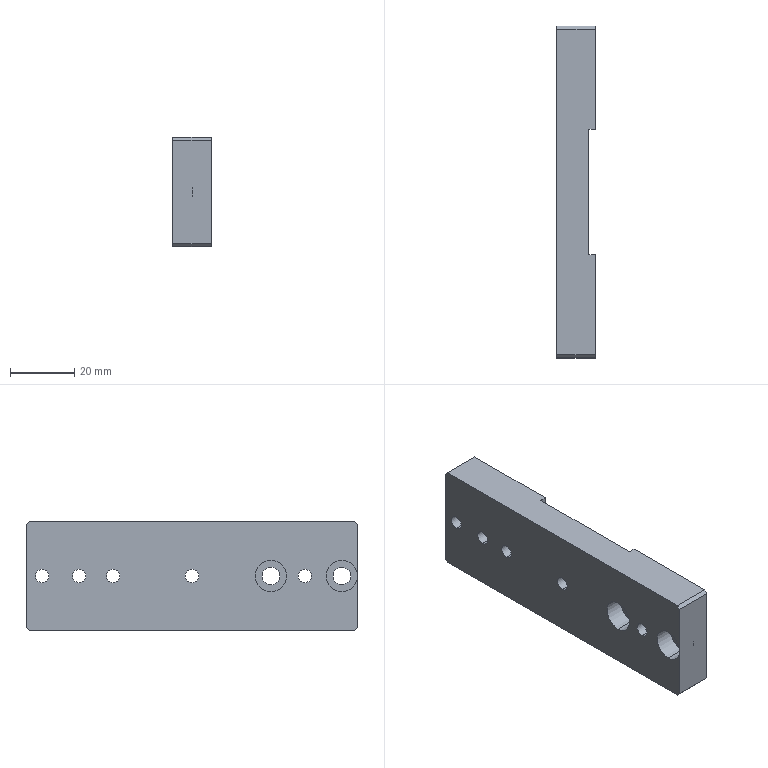Component | SolidWorks | MTCTV2104DJ006-000-0038Slider-1 | 1 solid | 34 faces | box 12 x 103 x 34 mm | volume 37354 mm3 | cylinder 18 | plane 16 | commonest cylinder face diameters 4.2 x10 9.8 x4 5.5 x4
STEP:
#1=COLOUR_RGB('',0.7922,0.8196,0.9333);
#2=FILL_AREA_STYLE_COLOUR('',#1);
#3=FILL_AREA_STYLE('',(#2));
#4=SURFACE_STYLE_FILL_AREA(#3);
#5=SURFACE_SIDE_STYLE('',(#4));
#6=SURFACE_STYLE_USAGE(.BOTH.,#5);
#7=PRESENTATION_STYLE_ASSIGNMENT((#6));
#8=CARTESIAN_POINT('',(1.803,-1.19,10.258));
#9=VERTEX_POINT('',#8);
#10=CARTESIAN_POINT('',(1.803,-1.19,10.644));
#11=VERTEX_POINT('',#10);
#12=CARTESIAN_POINT('',(1.803,-1.19,10.451));
#13=DIRECTION('',(-1.,-0.,-0.));
#14=DIRECTION('',(0.,0.,1.));
#15=AXIS2_PLACEMENT_3D('',#12,#13,#14);
#16=CIRCLE('',#15,0.1929);
#17=EDGE_CURVE('',#9,#11,#16,.T.);
#18=ORIENTED_EDGE('',*,*,#17,.F.);
#19=CARTESIAN_POINT('',(1.567,-1.19,10.258));
#20=VERTEX_POINT('',#19);
#21=CARTESIAN_POINT('',(1.567,-1.19,10.258));
#22=DIRECTION('',(-1.,-0.,-0.));
#23=VECTOR('',#22,39.37);
#24=LINE('',#21,#23);
#25=EDGE_CURVE('',#9,#20,#24,.T.);
#26=ORIENTED_EDGE('',*,*,#25,.T.);
#27=CARTESIAN_POINT('',(1.567,-1.19,10.644));
#28=VERTEX_POINT('',#27);
#29=CARTESIAN_POINT('',(1.567,-1.19,10.451));
#30=DIRECTION('',(-1.,-0.,-0.));
#31=DIRECTION('',(0.,0.,1.));
#32=AXIS2_PLACEMENT_3D('',#29,#30,#31);
#33=CIRCLE('',#32,0.1929);
#34=EDGE_CURVE('',#20,#28,#33,.T.);
#35=ORIENTED_EDGE('',*,*,#34,.T.);
#36=CARTESIAN_POINT('',(1.567,-1.19,10.644));
#37=DIRECTION('',(-1.,-0.,-0.));
#38=VECTOR('',#37,39.37);
#39=LINE('',#36,#38);
#40=EDGE_CURVE('',#11,#28,#39,.T.);
#41=ORIENTED_EDGE('',*,*,#40,.F.);
#42=EDGE_LOOP('',(#18,#26,#35,#41));
#43=FACE_OUTER_BOUND('',#42,.T.);
#44=CARTESIAN_POINT('',(1.567,-1.19,10.451));
#45=DIRECTION('',(-1.,-0.,-0.));
#46=DIRECTION('',(0.,0.,1.));
#47=AXIS2_PLACEMENT_3D('',#44,#45,#46);
#48=CYLINDRICAL_SURFACE('',#47,0.1929);
#49=ADVANCED_FACE('',(#43),#48,.F.);
#50=CARTESIAN_POINT('',(2.039,-1.19,10.559));
#51=VERTEX_POINT('',#50);
#52=CARTESIAN_POINT('',(2.039,-1.19,10.342));
#53=VERTEX_POINT('',#52);
#54=CARTESIAN_POINT('',(2.039,-1.19,10.451));
#55=DIRECTION('',(1.,0.,0.));
#56=DIRECTION('',(0.,0.,-1.));
#57=AXIS2_PLACEMENT_3D('',#54,#55,#56);
#58=CIRCLE('',#57,0.1083);
#59=EDGE_CURVE('',#51,#53,#58,.T.);
#60=ORIENTED_EDGE('',*,*,#59,.T.);
#61=CARTESIAN_POINT('',(1.803,-1.19,10.342));
#62=VERTEX_POINT('',#61);
#63=CARTESIAN_POINT('',(1.567,-1.19,10.342));
#64=DIRECTION('',(-1.,-0.,-0.));
#65=VECTOR('',#64,39.37);
#66=LINE('',#63,#65);
#67=EDGE_CURVE('',#53,#62,#66,.T.);
#68=ORIENTED_EDGE('',*,*,#67,.T.);
#69=CARTESIAN_POINT('',(1.803,-1.19,10.559));
#70=VERTEX_POINT('',#69);
#71=CARTESIAN_POINT('',(1.803,-1.19,10.451));
#72=DIRECTION('',(-1.,-0.,-0.));
#73=DIRECTION('',(0.,0.,1.));
#74=AXIS2_PLACEMENT_3D('',#71,#72,#73);
#75=CIRCLE('',#74,0.1083);
#76=EDGE_CURVE('',#62,#70,#75,.T.);
#77=ORIENTED_EDGE('',*,*,#76,.T.);
#78=CARTESIAN_POINT('',(1.567,-1.19,10.559));
#79=DIRECTION('',(-1.,-0.,-0.));
#80=VECTOR('',#79,39.37);
#81=LINE('',#78,#80);
#82=EDGE_CURVE('',#51,#70,#81,.T.);
#83=ORIENTED_EDGE('',*,*,#82,.F.);
#84=EDGE_LOOP('',(#60,#68,#77,#83));
#85=FACE_OUTER_BOUND('',#84,.T.);
#86=CARTESIAN_POINT('',(1.567,-1.19,10.451));
#87=DIRECTION('',(-1.,-0.,-0.));
#88=DIRECTION('',(0.,0.,1.));
#89=AXIS2_PLACEMENT_3D('',#86,#87,#88);
#90=CYLINDRICAL_SURFACE('',#89,0.1083);
#91=ADVANCED_FACE('',(#85),#90,.F.);
#92=CARTESIAN_POINT('',(1.803,-2.056,10.258));
#93=VERTEX_POINT('',#92);
#94=CARTESIAN_POINT('',(1.803,-2.056,10.644));
#95=VERTEX_POINT('',#94);
#96=CARTESIAN_POINT('',(1.803,-2.056,10.451));
#97=DIRECTION('',(-1.,-0.,-0.));
#98=DIRECTION('',(0.,0.,1.));
#99=AXIS2_PLACEMENT_3D('',#96,#97,#98);
#100=CIRCLE('',#99,0.1929);
#101=EDGE_CURVE('',#93,#95,#100,.T.);
#102=ORIENTED_EDGE('',*,*,#101,.F.);
#103=CARTESIAN_POINT('',(1.567,-2.056,10.258));
#104=VERTEX_POINT('',#103);
#105=CARTESIAN_POINT('',(1.567,-2.056,10.258));
#106=DIRECTION('',(-1.,-0.,-0.));
#107=VECTOR('',#106,39.37);
#108=LINE('',#105,#107);
#109=EDGE_CURVE('',#93,#104,#108,.T.);
#110=ORIENTED_EDGE('',*,*,#109,.T.);
#111=CARTESIAN_POINT('',(1.567,-2.056,10.644));
#112=VERTEX_POINT('',#111);
#113=CARTESIAN_POINT('',(1.567,-2.056,10.451));
#114=DIRECTION('',(-1.,-0.,-0.));
#115=DIRECTION('',(0.,0.,1.));
#116=AXIS2_PLACEMENT_3D('',#113,#114,#115);
#117=CIRCLE('',#116,0.1929);
#118=EDGE_CURVE('',#104,#112,#117,.T.);
#119=ORIENTED_EDGE('',*,*,#118,.T.);
#120=CARTESIAN_POINT('',(1.567,-2.056,10.644));
#121=DIRECTION('',(-1.,-0.,-0.));
#122=VECTOR('',#121,39.37);
#123=LINE('',#120,#122);
#124=EDGE_CURVE('',#95,#112,#123,.T.);
#125=ORIENTED_EDGE('',*,*,#124,.F.);
#126=EDGE_LOOP('',(#102,#110,#119,#125));
#127=FACE_OUTER_BOUND('',#126,.T.);
#128=CARTESIAN_POINT('',(1.567,-2.056,10.451));
#129=DIRECTION('',(-1.,-0.,-0.));
#130=DIRECTION('',(0.,0.,1.));
#131=AXIS2_PLACEMENT_3D('',#128,#129,#130);
#132=CYLINDRICAL_SURFACE('',#131,0.1929);
#133=ADVANCED_FACE('',(#127),#132,.F.);
#134=CARTESIAN_POINT('',(2.039,-2.056,10.559));
#135=VERTEX_POINT('',#134);
#136=CARTESIAN_POINT('',(2.039,-2.056,10.342));
#137=VERTEX_POINT('',#136);
#138=CARTESIAN_POINT('',(2.039,-2.056,10.451));
#139=DIRECTION('',(1.,0.,0.));
#140=DIRECTION('',(0.,0.,-1.));
#141=AXIS2_PLACEMENT_3D('',#138,#139,#140);
#142=CIRCLE('',#141,0.1083);
#143=EDGE_CURVE('',#135,#137,#142,.T.);
#144=ORIENTED_EDGE('',*,*,#143,.T.);
#145=CARTESIAN_POINT('',(1.803,-2.056,10.342));
#146=VERTEX_POINT('',#145);
#147=CARTESIAN_POINT('',(1.567,-2.056,10.342));
#148=DIRECTION('',(-1.,-0.,-0.));
#149=VECTOR('',#148,39.37);
#150=LINE('',#147,#149);
#151=EDGE_CURVE('',#137,#146,#150,.T.);
#152=ORIENTED_EDGE('',*,*,#151,.T.);
#153=CARTESIAN_POINT('',(1.803,-2.056,10.559));
#154=VERTEX_POINT('',#153);
#155=CARTESIAN_POINT('',(1.803,-2.056,10.451));
#156=DIRECTION('',(-1.,-0.,-0.));
#157=DIRECTION('',(0.,0.,1.));
#158=AXIS2_PLACEMENT_3D('',#155,#156,#157);
#159=CIRCLE('',#158,0.1083);
#160=EDGE_CURVE('',#146,#154,#159,.T.);
#161=ORIENTED_EDGE('',*,*,#160,.T.);
#162=CARTESIAN_POINT('',(1.567,-2.056,10.559));
#163=DIRECTION('',(-1.,-0.,-0.));
#164=VECTOR('',#163,39.37);
#165=LINE('',#162,#164);
#166=EDGE_CURVE('',#135,#154,#165,.T.);
#167=ORIENTED_EDGE('',*,*,#166,.F.);
#168=EDGE_LOOP('',(#144,#152,#161,#167));
#169=FACE_OUTER_BOUND('',#168,.T.);
#170=CARTESIAN_POINT('',(1.567,-2.056,10.451));
#171=DIRECTION('',(-1.,-0.,-0.));
#172=DIRECTION('',(0.,0.,1.));
#173=AXIS2_PLACEMENT_3D('',#170,#171,#172);
#174=CYLINDRICAL_SURFACE('',#173,0.1083);
#175=ADVANCED_FACE('',(#169),#174,.F.);
#176=CARTESIAN_POINT('',(2.039,1.153,10.533));
#177=VERTEX_POINT('',#176);
#178=CARTESIAN_POINT('',(2.039,1.153,10.368));
#179=VERTEX_POINT('',#178);
#180=CARTESIAN_POINT('',(2.039,1.153,10.451));
#181=DIRECTION('',(1.,0.,0.));
#182=DIRECTION('',(0.,0.,-1.));
#183=AXIS2_PLACEMENT_3D('',#180,#181,#182);
#184=CIRCLE('',#183,0.08268);
#185=EDGE_CURVE('',#177,#179,#184,.T.);
#186=ORIENTED_EDGE('',*,*,#185,.T.);
#187=CARTESIAN_POINT('',(1.567,1.153,10.368));
#188=VERTEX_POINT('',#187);
#189=CARTESIAN_POINT('',(1.567,1.153,10.368));
#190=DIRECTION('',(-1.,-0.,-0.));
#191=VECTOR('',#190,39.37);
#192=LINE('',#189,#191);
#193=EDGE_CURVE('',#179,#188,#192,.T.);
#194=ORIENTED_EDGE('',*,*,#193,.T.);
#195=CARTESIAN_POINT('',(1.567,1.153,10.533));
#196=VERTEX_POINT('',#195);
#197=CARTESIAN_POINT('',(1.567,1.153,10.451));
#198=DIRECTION('',(-1.,-0.,-0.));
#199=DIRECTION('',(0.,0.,1.));
#200=AXIS2_PLACEMENT_3D('',#197,#198,#199);
#201=CIRCLE('',#200,0.08268);
#202=EDGE_CURVE('',#188,#196,#201,.T.);
#203=ORIENTED_EDGE('',*,*,#202,.T.);
#204=CARTESIAN_POINT('',(1.567,1.153,10.533));
#205=DIRECTION('',(-1.,-0.,-0.));
#206=VECTOR('',#205,39.37);
#207=LINE('',#204,#206);
#208=EDGE_CURVE('',#177,#196,#207,.T.);
#209=ORIENTED_EDGE('',*,*,#208,.F.);
#210=EDGE_LOOP('',(#186,#194,#203,#209));
#211=FACE_OUTER_BOUND('',#210,.T.);
#212=CARTESIAN_POINT('',(1.567,1.153,10.451));
#213=DIRECTION('',(-1.,-0.,-0.));
#214=DIRECTION('',(0.,0.,1.));
#215=AXIS2_PLACEMENT_3D('',#212,#213,#214);
#216=CYLINDRICAL_SURFACE('',#215,0.08268);
#217=ADVANCED_FACE('',(#211),#216,.F.);
#218=CARTESIAN_POINT('',(2.039,-1.603,10.533));
#219=VERTEX_POINT('',#218);
#220=CARTESIAN_POINT('',(2.039,-1.603,10.368));
#221=VERTEX_POINT('',#220);
#222=CARTESIAN_POINT('',(2.039,-1.603,10.451));
#223=DIRECTION('',(1.,0.,0.));
#224=DIRECTION('',(0.,0.,-1.));
#225=AXIS2_PLACEMENT_3D('',#222,#223,#224);
#226=CIRCLE('',#225,0.08268);
#227=EDGE_CURVE('',#219,#221,#226,.T.);
#228=ORIENTED_EDGE('',*,*,#227,.T.);
#229=CARTESIAN_POINT('',(1.567,-1.603,10.368));
#230=VERTEX_POINT('',#229);
#231=CARTESIAN_POINT('',(1.567,-1.603,10.368));
#232=DIRECTION('',(-1.,-0.,-0.));
#233=VECTOR('',#232,39.37);
#234=LINE('',#231,#233);
#235=EDGE_CURVE('',#221,#230,#234,.T.);
#236=ORIENTED_EDGE('',*,*,#235,.T.);
#237=CARTESIAN_POINT('',(1.567,-1.603,10.533));
#238=VERTEX_POINT('',#237);
#239=CARTESIAN_POINT('',(1.567,-1.603,10.451));
#240=DIRECTION('',(-1.,-0.,-0.));
#241=DIRECTION('',(0.,0.,1.));
#242=AXIS2_PLACEMENT_3D('',#239,#240,#241);
#243=CIRCLE('',#242,0.08268);
#244=EDGE_CURVE('',#230,#238,#243,.T.);
#245=ORIENTED_EDGE('',*,*,#244,.T.);
#246=CARTESIAN_POINT('',(1.567,-1.603,10.533));
#247=DIRECTION('',(-1.,-0.,-0.));
#248=VECTOR('',#247,39.37);
#249=LINE('',#246,#248);
#250=EDGE_CURVE('',#219,#238,#249,.T.);
#251=ORIENTED_EDGE('',*,*,#250,.F.);
#252=EDGE_LOOP('',(#228,#236,#245,#251));
#253=FACE_OUTER_BOUND('',#252,.T.);
#254=CARTESIAN_POINT('',(1.567,-1.603,10.451));
#255=DIRECTION('',(-1.,-0.,-0.));
#256=DIRECTION('',(0.,0.,1.));
#257=AXIS2_PLACEMENT_3D('',#254,#255,#256);
#258=CYLINDRICAL_SURFACE('',#257,0.08268);
#259=ADVANCED_FACE('',(#253),#258,.F.);
#260=CARTESIAN_POINT('',(1.961,-0.2251,10.368));
#261=VERTEX_POINT('',#260);
#262=CARTESIAN_POINT('',(1.961,-0.2251,10.533));
#263=VERTEX_POINT('',#262);
#264=CARTESIAN_POINT('',(1.961,-0.2251,10.451));
#265=DIRECTION('',(-1.,-0.,-0.));
#266=DIRECTION('',(0.,0.,1.));
#267=AXIS2_PLACEMENT_3D('',#264,#265,#266);
#268=CIRCLE('',#267,0.08268);
#269=EDGE_CURVE('',#261,#263,#268,.T.);
#270=ORIENTED_EDGE('',*,*,#269,.F.);
#271=CARTESIAN_POINT('',(1.567,-0.2251,10.368));
#272=VERTEX_POINT('',#271);
#273=CARTESIAN_POINT('',(1.567,-0.2251,10.368));
#274=DIRECTION('',(-1.,-0.,-0.));
#275=VECTOR('',#274,39.37);
#276=LINE('',#273,#275);
#277=EDGE_CURVE('',#261,#272,#276,.T.);
#278=ORIENTED_EDGE('',*,*,#277,.T.);
#279=CARTESIAN_POINT('',(1.567,-0.2251,10.533));
#280=VERTEX_POINT('',#279);
#281=CARTESIAN_POINT('',(1.567,-0.2251,10.451));
#282=DIRECTION('',(-1.,-0.,-0.));
#283=DIRECTION('',(0.,0.,1.));
#284=AXIS2_PLACEMENT_3D('',#281,#282,#283);
#285=CIRCLE('',#284,0.08268);
#286=EDGE_CURVE('',#272,#280,#285,.T.);
#287=ORIENTED_EDGE('',*,*,#286,.T.);
#288=CARTESIAN_POINT('',(1.567,-0.2251,10.533));
#289=DIRECTION('',(-1.,-0.,-0.));
#290=VECTOR('',#289,39.37);
#291=LINE('',#288,#290);
#292=EDGE_CURVE('',#263,#280,#291,.T.);
#293=ORIENTED_EDGE('',*,*,#292,.F.);
#294=EDGE_LOOP('',(#270,#278,#287,#293));
#295=FACE_OUTER_BOUND('',#294,.T.);
#296=CARTESIAN_POINT('',(1.567,-0.2251,10.451));
#297=DIRECTION('',(-1.,-0.,-0.));
#298=DIRECTION('',(0.,0.,1.));
#299=AXIS2_PLACEMENT_3D('',#296,#297,#298);
#300=CYLINDRICAL_SURFACE('',#299,0.08268);
#301=ADVANCED_FACE('',(#295),#300,.F.);
#302=CARTESIAN_POINT('',(2.039,1.606,10.533));
#303=VERTEX_POINT('',#302);
#304=CARTESIAN_POINT('',(2.039,1.606,10.368));
#305=VERTEX_POINT('',#304);
#306=CARTESIAN_POINT('',(2.039,1.606,10.451));
#307=DIRECTION('',(1.,0.,0.));
#308=DIRECTION('',(0.,0.,-1.));
#309=AXIS2_PLACEMENT_3D('',#306,#307,#308);
#310=CIRCLE('',#309,0.08268);
#311=EDGE_CURVE('',#303,#305,#310,.T.);
#312=ORIENTED_EDGE('',*,*,#311,.T.);
#313=CARTESIAN_POINT('',(1.567,1.606,10.368));
#314=VERTEX_POINT('',#313);
#315=CARTESIAN_POINT('',(1.567,1.606,10.368));
#316=DIRECTION('',(-1.,-0.,-0.));
#317=VECTOR('',#316,39.37);
#318=LINE('',#315,#317);
#319=EDGE_CURVE('',#305,#314,#318,.T.);
#320=ORIENTED_EDGE('',*,*,#319,.T.);
#321=CARTESIAN_POINT('',(1.567,1.606,10.533));
#322=VERTEX_POINT('',#321);
#323=CARTESIAN_POINT('',(1.567,1.606,10.451));
#324=DIRECTION('',(-1.,-0.,-0.));
#325=DIRECTION('',(0.,0.,1.));
#326=AXIS2_PLACEMENT_3D('',#323,#324,#325);
#327=CIRCLE('',#326,0.08268);
#328=EDGE_CURVE('',#314,#322,#327,.T.);
#329=ORIENTED_EDGE('',*,*,#328,.T.);
#330=CARTESIAN_POINT('',(1.567,1.606,10.533));
#331=DIRECTION('',(-1.,-0.,-0.));
#332=VECTOR('',#331,39.37);
#333=LINE('',#330,#332);
#334=EDGE_CURVE('',#303,#322,#333,.T.);
#335=ORIENTED_EDGE('',*,*,#334,.F.);
#336=EDGE_LOOP('',(#312,#320,#329,#335));
#337=FACE_OUTER_BOUND('',#336,.T.);
#338=CARTESIAN_POINT('',(1.567,1.606,10.451));
#339=DIRECTION('',(-1.,-0.,-0.));
#340=DIRECTION('',(0.,0.,1.));
#341=AXIS2_PLACEMENT_3D('',#338,#339,#340);
#342=CYLINDRICAL_SURFACE('',#341,0.08268);
#343=ADVANCED_FACE('',(#337),#342,.F.);
#344=CARTESIAN_POINT('',(2.039,0.7394,10.533));
#345=VERTEX_POINT('',#344);
#346=CARTESIAN_POINT('',(2.039,0.7394,10.368));
#347=VERTEX_POINT('',#346);
#348=CARTESIAN_POINT('',(2.039,0.7394,10.451));
#349=DIRECTION('',(1.,0.,0.));
#350=DIRECTION('',(0.,0.,-1.));
#351=AXIS2_PLACEMENT_3D('',#348,#349,#350);
#352=CIRCLE('',#351,0.08268);
#353=EDGE_CURVE('',#345,#347,#352,.T.);
#354=ORIENTED_EDGE('',*,*,#353,.T.);
#355=CARTESIAN_POINT('',(1.567,0.7394,10.368));
#356=VERTEX_POINT('',#355);
#357=CARTESIAN_POINT('',(1.567,0.7394,10.368));
#358=DIRECTION('',(-1.,-0.,-0.));
#359=VECTOR('',#358,39.37);
#360=LINE('',#357,#359);
#361=EDGE_CURVE('',#347,#356,#360,.T.);
#362=ORIENTED_EDGE('',*,*,#361,.T.);
#363=CARTESIAN_POINT('',(1.567,0.7394,10.533));
#364=VERTEX_POINT('',#363);
#365=CARTESIAN_POINT('',(1.567,0.7394,10.451));
#366=DIRECTION('',(-1.,-0.,-0.));
#367=DIRECTION('',(0.,0.,1.));
#368=AXIS2_PLACEMENT_3D('',#365,#366,#367);
#369=CIRCLE('',#368,0.08268);
#370=EDGE_CURVE('',#356,#364,#369,.T.);
#371=ORIENTED_EDGE('',*,*,#370,.T.);
#372=CARTESIAN_POINT('',(1.567,0.7394,10.533));
#373=DIRECTION('',(-1.,-0.,-0.));
#374=VECTOR('',#373,39.37);
#375=LINE('',#372,#374);
#376=EDGE_CURVE('',#345,#364,#375,.T.);
#377=ORIENTED_EDGE('',*,*,#376,.F.);
#378=EDGE_LOOP('',(#354,#362,#371,#377));
#379=FACE_OUTER_BOUND('',#378,.T.);
#380=CARTESIAN_POINT('',(1.567,0.7394,10.451));
#381=DIRECTION('',(-1.,-0.,-0.));
#382=DIRECTION('',(0.,0.,1.));
#383=AXIS2_PLACEMENT_3D('',#380,#381,#382);
#384=CYLINDRICAL_SURFACE('',#383,0.08268);
#385=ADVANCED_FACE('',(#379),#384,.F.);
#386=CARTESIAN_POINT('',(1.961,-0.2251,10.451));
#387=DIRECTION('',(-1.,-0.,-0.));
#388=DIRECTION('',(0.,0.,1.));
#389=AXIS2_PLACEMENT_3D('',#386,#387,#388);
#390=CIRCLE('',#389,0.08268);
#391=EDGE_CURVE('',#263,#261,#390,.T.);
#392=ORIENTED_EDGE('',*,*,#391,.T.);
#393=ORIENTED_EDGE('',*,*,#269,.T.);
#394=EDGE_LOOP('',(#392,#393));
#395=FACE_BOUND('',#394,.T.);
#396=CARTESIAN_POINT('',(1.961,-0.9929,11.12));
#397=VERTEX_POINT('',#396);
#398=CARTESIAN_POINT('',(1.961,0.5426,11.12));
#399=VERTEX_POINT('',#398);
#400=CARTESIAN_POINT('',(1.961,-2.253,11.12));
#401=DIRECTION('',(-0.,1.,0.));
#402=VECTOR('',#401,39.37);
#403=LINE('',#400,#402);
#404=EDGE_CURVE('',#397,#399,#403,.T.);
#405=ORIENTED_EDGE('',*,*,#404,.F.);
#406=CARTESIAN_POINT('',(1.961,-0.9929,9.781));
#407=VERTEX_POINT('',#406);
#408=CARTESIAN_POINT('',(1.961,-0.9929,11.12));
#409=DIRECTION('',(-0.,-0.,1.));
#410=VECTOR('',#409,39.37);
#411=LINE('',#408,#410);
#412=EDGE_CURVE('',#407,#397,#411,.T.);
#413=ORIENTED_EDGE('',*,*,#412,.F.);
#414=CARTESIAN_POINT('',(1.961,0.5426,9.781));
#415=VERTEX_POINT('',#414);
#416=CARTESIAN_POINT('',(1.961,-2.253,9.781));
#417=DIRECTION('',(0.,-1.,-0.));
#418=VECTOR('',#417,39.37);
#419=LINE('',#416,#418);
#420=EDGE_CURVE('',#415,#407,#419,.T.);
#421=ORIENTED_EDGE('',*,*,#420,.F.);
#422=CARTESIAN_POINT('',(1.961,0.5426,11.12));
#423=DIRECTION('',(0.,0.,-1.));
#424=VECTOR('',#423,39.37);
#425=LINE('',#422,#424);
#426=EDGE_CURVE('',#399,#415,#425,.T.);
#427=ORIENTED_EDGE('',*,*,#426,.F.);
#428=EDGE_LOOP('',(#405,#413,#421,#427));
#429=FACE_OUTER_BOUND('',#428,.T.);
#430=CARTESIAN_POINT('',(1.961,-0.2251,10.451));
#431=DIRECTION('',(1.,0.,0.));
#432=DIRECTION('',(0.,0.,-1.));
#433=AXIS2_PLACEMENT_3D('',#430,#431,#432);
#434=PLANE('',#433);
#435=ADVANCED_FACE('',(#395,#429),#434,.T.);
#436=CARTESIAN_POINT('',(1.567,-1.19,10.451));
#437=DIRECTION('',(-1.,-0.,-0.));
#438=DIRECTION('',(0.,0.,1.));
#439=AXIS2_PLACEMENT_3D('',#436,#437,#438);
#440=CIRCLE('',#439,0.1929);
#441=EDGE_CURVE('',#28,#20,#440,.T.);
#442=ORIENTED_EDGE('',*,*,#441,.F.);
#443=ORIENTED_EDGE('',*,*,#34,.F.);
#444=EDGE_LOOP('',(#442,#443));
#445=FACE_BOUND('',#444,.T.);
#446=CARTESIAN_POINT('',(1.567,-2.253,9.821));
#447=VERTEX_POINT('',#446);
#448=CARTESIAN_POINT('',(1.567,-2.253,11.081));
#449=VERTEX_POINT('',#448);
#450=CARTESIAN_POINT('',(1.567,-2.253,9.781));
#451=DIRECTION('',(-0.,-0.,1.));
#452=VECTOR('',#451,39.37);
#453=LINE('',#450,#452);
#454=EDGE_CURVE('',#447,#449,#453,.T.);
#455=ORIENTED_EDGE('',*,*,#454,.T.);
#456=CARTESIAN_POINT('',(1.567,-2.213,11.12));
#457=VERTEX_POINT('',#456);
#458=CARTESIAN_POINT('',(1.567,-2.213,11.12));
#459=DIRECTION('',(-0.,0.7071,0.7071));
#460=VECTOR('',#459,39.37);
#461=LINE('',#458,#460);
#462=EDGE_CURVE('',#449,#457,#461,.T.);
#463=ORIENTED_EDGE('',*,*,#462,.T.);
#464=CARTESIAN_POINT('',(1.567,1.763,11.12));
#465=VERTEX_POINT('',#464);
#466=CARTESIAN_POINT('',(1.567,-2.253,11.12));
#467=DIRECTION('',(-0.,1.,0.));
#468=VECTOR('',#467,39.37);
#469=LINE('',#466,#468);
#470=EDGE_CURVE('',#457,#465,#469,.T.);
#471=ORIENTED_EDGE('',*,*,#470,.T.);
#472=CARTESIAN_POINT('',(1.567,1.802,11.081));
#473=VERTEX_POINT('',#472);
#474=CARTESIAN_POINT('',(1.567,1.802,11.081));
#475=DIRECTION('',(-0.,0.7071,-0.7071));
#476=VECTOR('',#475,39.37);
#477=LINE('',#474,#476);
#478=EDGE_CURVE('',#465,#473,#477,.T.);
#479=ORIENTED_EDGE('',*,*,#478,.T.);
#480=CARTESIAN_POINT('',(1.567,1.802,9.821));
#481=VERTEX_POINT('',#480);
#482=CARTESIAN_POINT('',(1.567,1.802,9.781));
#483=DIRECTION('',(0.,0.,-1.));
#484=VECTOR('',#483,39.37);
#485=LINE('',#482,#484);
#486=EDGE_CURVE('',#473,#481,#485,.T.);
#487=ORIENTED_EDGE('',*,*,#486,.T.);
#488=CARTESIAN_POINT('',(1.567,1.763,9.781));
#489=VERTEX_POINT('',#488);
#490=CARTESIAN_POINT('',(1.567,1.763,9.781));
#491=DIRECTION('',(0.,-0.7071,-0.7071));
#492=VECTOR('',#491,39.37);
#493=LINE('',#490,#492);
#494=EDGE_CURVE('',#481,#489,#493,.T.);
#495=ORIENTED_EDGE('',*,*,#494,.T.);
#496=CARTESIAN_POINT('',(1.567,-2.213,9.781));
#497=VERTEX_POINT('',#496);
#498=CARTESIAN_POINT('',(1.567,-2.253,9.781));
#499=DIRECTION('',(0.,-1.,-0.));
#500=VECTOR('',#499,39.37);
#501=LINE('',#498,#500);
#502=EDGE_CURVE('',#489,#497,#501,.T.);
#503=ORIENTED_EDGE('',*,*,#502,.T.);
#504=CARTESIAN_POINT('',(1.567,-2.253,9.821));
#505=DIRECTION('',(0.,-0.7071,0.7071));
#506=VECTOR('',#505,39.37);
#507=LINE('',#504,#506);
#508=EDGE_CURVE('',#497,#447,#507,.T.);
#509=ORIENTED_EDGE('',*,*,#508,.T.);
#510=EDGE_LOOP('',(#455,#463,#471,#479,#487,#495,#503,#509));
#511=FACE_OUTER_BOUND('',#510,.T.);
#512=CARTESIAN_POINT('',(1.567,0.7394,10.451));
#513=DIRECTION('',(-1.,-0.,-0.));
#514=DIRECTION('',(0.,0.,1.));
#515=AXIS2_PLACEMENT_3D('',#512,#513,#514);
#516=CIRCLE('',#515,0.08268);
#517=EDGE_CURVE('',#364,#356,#516,.T.);
#518=ORIENTED_EDGE('',*,*,#517,.F.);
#519=ORIENTED_EDGE('',*,*,#370,.F.);
#520=EDGE_LOOP('',(#518,#519));
#521=FACE_BOUND('',#520,.T.);
#522=CARTESIAN_POINT('',(1.567,1.606,10.451));
#523=DIRECTION('',(-1.,-0.,-0.));
#524=DIRECTION('',(0.,0.,1.));
#525=AXIS2_PLACEMENT_3D('',#522,#523,#524);
#526=CIRCLE('',#525,0.08268);
#527=EDGE_CURVE('',#322,#314,#526,.T.);
#528=ORIENTED_EDGE('',*,*,#527,.F.);
#529=ORIENTED_EDGE('',*,*,#328,.F.);
#530=EDGE_LOOP('',(#528,#529));
#531=FACE_BOUND('',#530,.T.);
#532=CARTESIAN_POINT('',(1.567,-0.2251,10.451));
#533=DIRECTION('',(-1.,-0.,-0.));
#534=DIRECTION('',(0.,0.,1.));
#535=AXIS2_PLACEMENT_3D('',#532,#533,#534);
#536=CIRCLE('',#535,0.08268);
#537=EDGE_CURVE('',#280,#272,#536,.T.);
#538=ORIENTED_EDGE('',*,*,#537,.F.);
#539=ORIENTED_EDGE('',*,*,#286,.F.);
#540=EDGE_LOOP('',(#538,#539));
#541=FACE_BOUND('',#540,.T.);
#542=CARTESIAN_POINT('',(1.567,-1.603,10.451));
#543=DIRECTION('',(-1.,-0.,-0.));
#544=DIRECTION('',(0.,0.,1.));
#545=AXIS2_PLACEMENT_3D('',#542,#543,#544);
#546=CIRCLE('',#545,0.08268);
#547=EDGE_CURVE('',#238,#230,#546,.T.);
#548=ORIENTED_EDGE('',*,*,#547,.F.);
#549=ORIENTED_EDGE('',*,*,#244,.F.);
#550=EDGE_LOOP('',(#548,#549));
#551=FACE_BOUND('',#550,.T.);
#552=CARTESIAN_POINT('',(1.567,1.153,10.451));
#553=DIRECTION('',(-1.,-0.,-0.));
#554=DIRECTION('',(0.,0.,1.));
#555=AXIS2_PLACEMENT_3D('',#552,#553,#554);
#556=CIRCLE('',#555,0.08268);
#557=EDGE_CURVE('',#196,#188,#556,.T.);
#558=ORIENTED_EDGE('',*,*,#557,.F.);
#559=ORIENTED_EDGE('',*,*,#202,.F.);
#560=EDGE_LOOP('',(#558,#559));
#561=FACE_BOUND('',#560,.T.);
#562=CARTESIAN_POINT('',(1.567,-2.056,10.451));
#563=DIRECTION('',(-1.,-0.,-0.));
#564=DIRECTION('',(0.,0.,1.));
#565=AXIS2_PLACEMENT_3D('',#562,#563,#564);
#566=CIRCLE('',#565,0.1929);
#567=EDGE_CURVE('',#112,#104,#566,.T.);
#568=ORIENTED_EDGE('',*,*,#567,.F.);
#569=ORIENTED_EDGE('',*,*,#118,.F.);
#570=EDGE_LOOP('',(#568,#569));
#571=FACE_BOUND('',#570,.T.);
#572=CARTESIAN_POINT('',(1.567,-0.2251,10.451));
#573=DIRECTION('',(1.,0.,0.));
#574=DIRECTION('',(0.,0.,-1.));
#575=AXIS2_PLACEMENT_3D('',#572,#573,#574);
#576=PLANE('',#575);
#577=ADVANCED_FACE('',(#445,#511,#521,#531,#541,#551,#561,#571),#576,.F.);
#578=ORIENTED_EDGE('',*,*,#470,.F.);
#579=CARTESIAN_POINT('',(2.039,-2.213,11.12));
#580=VERTEX_POINT('',#579);
#581=CARTESIAN_POINT('',(1.567,-2.213,11.12));
#582=DIRECTION('',(1.,0.,0.));
#583=VECTOR('',#582,39.37);
#584=LINE('',#581,#583);
#585=EDGE_CURVE('',#457,#580,#584,.T.);
#586=ORIENTED_EDGE('',*,*,#585,.T.);
#587=CARTESIAN_POINT('',(2.039,-0.9929,11.12));
#588=VERTEX_POINT('',#587);
#589=CARTESIAN_POINT('',(2.039,-0.9929,11.12));
#590=DIRECTION('',(0.,-1.,-0.));
#591=VECTOR('',#590,39.37);
#592=LINE('',#589,#591);
#593=EDGE_CURVE('',#588,#580,#592,.T.);
#594=ORIENTED_EDGE('',*,*,#593,.F.);
#595=CARTESIAN_POINT('',(2.039,-0.9929,11.12));
#596=DIRECTION('',(-1.,-0.,-0.));
#597=VECTOR('',#596,39.37);
#598=LINE('',#595,#597);
#599=EDGE_CURVE('',#588,#397,#598,.T.);
#600=ORIENTED_EDGE('',*,*,#599,.T.);
#601=ORIENTED_EDGE('',*,*,#404,.T.);
#602=CARTESIAN_POINT('',(2.039,0.5426,11.12));
#603=VERTEX_POINT('',#602);
#604=CARTESIAN_POINT('',(2.039,0.5426,11.12));
#605=DIRECTION('',(-1.,-0.,-0.));
#606=VECTOR('',#605,39.37);
#607=LINE('',#604,#606);
#608=EDGE_CURVE('',#603,#399,#607,.T.);
#609=ORIENTED_EDGE('',*,*,#608,.F.);
#610=CARTESIAN_POINT('',(2.039,1.763,11.12));
#611=VERTEX_POINT('',#610);
#612=CARTESIAN_POINT('',(2.039,1.763,11.12));
#613=DIRECTION('',(0.,-1.,0.));
#614=VECTOR('',#613,39.37);
#615=LINE('',#612,#614);
#616=EDGE_CURVE('',#611,#603,#615,.T.);
#617=ORIENTED_EDGE('',*,*,#616,.F.);
#618=CARTESIAN_POINT('',(1.567,1.763,11.12));
#619=DIRECTION('',(-1.,-0.,-0.));
#620=VECTOR('',#619,39.37);
#621=LINE('',#618,#620);
#622=EDGE_CURVE('',#611,#465,#621,.T.);
#623=ORIENTED_EDGE('',*,*,#622,.T.);
#624=EDGE_LOOP('',(#578,#586,#594,#600,#601,#609,#617,#623));
#625=FACE_OUTER_BOUND('',#624,.T.);
#626=CARTESIAN_POINT('',(1.567,-2.253,11.12));
#627=DIRECTION('',(0.,0.,-1.));
#628=DIRECTION('',(-1.,-0.,-0.));
#629=AXIS2_PLACEMENT_3D('',#626,#627,#628);
#630=PLANE('',#629);
#631=ADVANCED_FACE('',(#625),#630,.F.);
#632=ORIENTED_EDGE('',*,*,#486,.F.);
#633=CARTESIAN_POINT('',(2.039,1.802,11.081));
#634=VERTEX_POINT('',#633);
#635=CARTESIAN_POINT('',(1.567,1.802,11.081));
#636=DIRECTION('',(1.,0.,0.));
#637=VECTOR('',#636,39.37);
#638=LINE('',#635,#637);
#639=EDGE_CURVE('',#473,#634,#638,.T.);
#640=ORIENTED_EDGE('',*,*,#639,.T.);
#641=CARTESIAN_POINT('',(2.039,1.802,9.821));
#642=VERTEX_POINT('',#641);
#643=CARTESIAN_POINT('',(2.039,1.802,9.821));
#644=DIRECTION('',(-0.,-0.,1.));
#645=VECTOR('',#644,39.37);
#646=LINE('',#643,#645);
#647=EDGE_CURVE('',#642,#634,#646,.T.);
#648=ORIENTED_EDGE('',*,*,#647,.F.);
#649=CARTESIAN_POINT('',(1.567,1.802,9.821));
#650=DIRECTION('',(-1.,-0.,-0.));
#651=VECTOR('',#650,39.37);
#652=LINE('',#649,#651);
#653=EDGE_CURVE('',#642,#481,#652,.T.);
#654=ORIENTED_EDGE('',*,*,#653,.T.);
#655=EDGE_LOOP('',(#632,#640,#648,#654));
#656=FACE_OUTER_BOUND('',#655,.T.);
#657=CARTESIAN_POINT('',(1.567,1.802,9.781));
#658=DIRECTION('',(0.,-1.,-0.));
#659=DIRECTION('',(-0.,-0.,1.));
#660=AXIS2_PLACEMENT_3D('',#657,#658,#659);
#661=PLANE('',#660);
#662=ADVANCED_FACE('',(#656),#661,.F.);
#663=CARTESIAN_POINT('',(2.039,1.763,9.781));
#664=VERTEX_POINT('',#663);
#665=CARTESIAN_POINT('',(1.567,1.763,9.781));
#666=DIRECTION('',(1.,0.,0.));
#667=VECTOR('',#666,39.37);
#668=LINE('',#665,#667);
#669=EDGE_CURVE('',#489,#664,#668,.T.);
#670=ORIENTED_EDGE('',*,*,#669,.T.);
#671=CARTESIAN_POINT('',(2.039,0.5426,9.781));
#672=VERTEX_POINT('',#671);
#673=CARTESIAN_POINT('',(2.039,0.5426,9.781));
#674=DIRECTION('',(-0.,1.,0.));
#675=VECTOR('',#674,39.37);
#676=LINE('',#673,#675);
#677=EDGE_CURVE('',#672,#664,#676,.T.);
#678=ORIENTED_EDGE('',*,*,#677,.F.);
#679=CARTESIAN_POINT('',(2.039,0.5426,9.781));
#680=DIRECTION('',(-1.,-0.,-0.));
#681=VECTOR('',#680,39.37);
#682=LINE('',#679,#681);
#683=EDGE_CURVE('',#672,#415,#682,.T.);
#684=ORIENTED_EDGE('',*,*,#683,.T.);
#685=ORIENTED_EDGE('',*,*,#420,.T.);
#686=CARTESIAN_POINT('',(2.039,-0.9929,9.781));
#687=VERTEX_POINT('',#686);
#688=CARTESIAN_POINT('',(2.039,-0.9929,9.781));
#689=DIRECTION('',(-1.,-0.,-0.));
#690=VECTOR('',#689,39.37);
#691=LINE('',#688,#690);
#692=EDGE_CURVE('',#687,#407,#691,.T.);
#693=ORIENTED_EDGE('',*,*,#692,.F.);
#694=CARTESIAN_POINT('',(2.039,-2.213,9.781));
#695=VERTEX_POINT('',#694);
#696=CARTESIAN_POINT('',(2.039,-2.213,9.781));
#697=DIRECTION('',(-0.,1.,0.));
#698=VECTOR('',#697,39.37);
#699=LINE('',#696,#698);
#700=EDGE_CURVE('',#695,#687,#699,.T.);
#701=ORIENTED_EDGE('',*,*,#700,.F.);
#702=CARTESIAN_POINT('',(1.567,-2.213,9.781));
#703=DIRECTION('',(-1.,-0.,-0.));
#704=VECTOR('',#703,39.37);
#705=LINE('',#702,#704);
#706=EDGE_CURVE('',#695,#497,#705,.T.);
#707=ORIENTED_EDGE('',*,*,#706,.T.);
#708=ORIENTED_EDGE('',*,*,#502,.F.);
#709=EDGE_LOOP('',(#670,#678,#684,#685,#693,#701,#707,#708));
#710=FACE_OUTER_BOUND('',#709,.T.);
#711=CARTESIAN_POINT('',(1.567,-2.253,9.781));
#712=DIRECTION('',(-0.,-0.,1.));
#713=DIRECTION('',(1.,0.,0.));
#714=AXIS2_PLACEMENT_3D('',#711,#712,#713);
#715=PLANE('',#714);
#716=ADVANCED_FACE('',(#710),#715,.F.);
#717=CARTESIAN_POINT('',(2.039,-2.253,9.821));
#718=VERTEX_POINT('',#717);
#719=CARTESIAN_POINT('',(1.567,-2.253,9.821));
#720=DIRECTION('',(1.,0.,0.));
#721=VECTOR('',#720,39.37);
#722=LINE('',#719,#721);
#723=EDGE_CURVE('',#447,#718,#722,.T.);
#724=ORIENTED_EDGE('',*,*,#723,.T.);
#725=CARTESIAN_POINT('',(2.039,-2.253,11.081));
#726=VERTEX_POINT('',#725);
#727=CARTESIAN_POINT('',(2.039,-2.253,11.081));
#728=DIRECTION('',(0.,0.,-1.));
#729=VECTOR('',#728,39.37);
#730=LINE('',#727,#729);
#731=EDGE_CURVE('',#726,#718,#730,.T.);
#732=ORIENTED_EDGE('',*,*,#731,.F.);
#733=CARTESIAN_POINT('',(1.567,-2.253,11.081));
#734=DIRECTION('',(-1.,-0.,-0.));
#735=VECTOR('',#734,39.37);
#736=LINE('',#733,#735);
#737=EDGE_CURVE('',#726,#449,#736,.T.);
#738=ORIENTED_EDGE('',*,*,#737,.T.);
#739=ORIENTED_EDGE('',*,*,#454,.F.);
#740=EDGE_LOOP('',(#724,#732,#738,#739));
#741=FACE_OUTER_BOUND('',#740,.T.);
#742=CARTESIAN_POINT('',(1.567,-2.253,9.781));
#743=DIRECTION('',(-0.,1.,0.));
#744=DIRECTION('',(0.,0.,-1.));
#745=AXIS2_PLACEMENT_3D('',#742,#743,#744);
#746=PLANE('',#745);
#747=ADVANCED_FACE('',(#741),#746,.F.);
#748=ORIENTED_EDGE('',*,*,#361,.F.);
#749=CARTESIAN_POINT('',(2.039,0.7394,10.451));
#750=DIRECTION('',(1.,0.,0.));
#751=DIRECTION('',(0.,0.,-1.));
#752=AXIS2_PLACEMENT_3D('',#749,#750,#751);
#753=CIRCLE('',#752,0.08268);
#754=EDGE_CURVE('',#347,#345,#753,.T.);
#755=ORIENTED_EDGE('',*,*,#754,.T.);
#756=ORIENTED_EDGE('',*,*,#376,.T.);
#757=ORIENTED_EDGE('',*,*,#517,.T.);
#758=EDGE_LOOP('',(#748,#755,#756,#757));
#759=FACE_OUTER_BOUND('',#758,.T.);
#760=CARTESIAN_POINT('',(1.567,0.7394,10.451));
#761=DIRECTION('',(-1.,-0.,-0.));
#762=DIRECTION('',(0.,0.,1.));
#763=AXIS2_PLACEMENT_3D('',#760,#761,#762);
#764=CYLINDRICAL_SURFACE('',#763,0.08268);
#765=ADVANCED_FACE('',(#759),#764,.F.);
#766=ORIENTED_EDGE('',*,*,#319,.F.);
#767=CARTESIAN_POINT('',(2.039,1.606,10.451));
#768=DIRECTION('',(1.,0.,0.));
#769=DIRECTION('',(0.,0.,-1.));
#770=AXIS2_PLACEMENT_3D('',#767,#768,#769);
#771=CIRCLE('',#770,0.08268);
#772=EDGE_CURVE('',#305,#303,#771,.T.);
#773=ORIENTED_EDGE('',*,*,#772,.T.);
#774=ORIENTED_EDGE('',*,*,#334,.T.);
#775=ORIENTED_EDGE('',*,*,#527,.T.);
#776=EDGE_LOOP('',(#766,#773,#774,#775));
#777=FACE_OUTER_BOUND('',#776,.T.);
#778=CARTESIAN_POINT('',(1.567,1.606,10.451));
#779=DIRECTION('',(-1.,-0.,-0.));
#780=DIRECTION('',(0.,0.,1.));
#781=AXIS2_PLACEMENT_3D('',#778,#779,#780);
#782=CYLINDRICAL_SURFACE('',#781,0.08268);
#783=ADVANCED_FACE('',(#777),#782,.F.);
#784=ORIENTED_EDGE('',*,*,#462,.F.);
#785=ORIENTED_EDGE('',*,*,#737,.F.);
#786=CARTESIAN_POINT('',(2.039,-2.213,11.12));
#787=DIRECTION('',(0.,-0.7071,-0.7071));
#788=VECTOR('',#787,39.37);
#789=LINE('',#786,#788);
#790=EDGE_CURVE('',#580,#726,#789,.T.);
#791=ORIENTED_EDGE('',*,*,#790,.F.);
#792=ORIENTED_EDGE('',*,*,#585,.F.);
#793=EDGE_LOOP('',(#784,#785,#791,#792));
#794=FACE_OUTER_BOUND('',#793,.T.);
#795=CARTESIAN_POINT('',(1.567,-2.213,11.12));
#796=DIRECTION('',(-0.,0.7071,-0.7071));
#797=DIRECTION('',(1.,0.,0.));
#798=AXIS2_PLACEMENT_3D('',#795,#796,#797);
#799=PLANE('',#798);
#800=ADVANCED_FACE('',(#794),#799,.F.);
#801=ORIENTED_EDGE('',*,*,#508,.F.);
#802=ORIENTED_EDGE('',*,*,#706,.F.);
#803=CARTESIAN_POINT('',(2.039,-2.253,9.821));
#804=DIRECTION('',(-0.,0.7071,-0.7071));
#805=VECTOR('',#804,39.37);
#806=LINE('',#803,#805);
#807=EDGE_CURVE('',#718,#695,#806,.T.);
#808=ORIENTED_EDGE('',*,*,#807,.F.);
#809=ORIENTED_EDGE('',*,*,#723,.F.);
#810=EDGE_LOOP('',(#801,#802,#808,#809));
#811=FACE_OUTER_BOUND('',#810,.T.);
#812=CARTESIAN_POINT('',(1.567,-2.253,9.821));
#813=DIRECTION('',(-0.,0.7071,0.7071));
#814=DIRECTION('',(1.,0.,0.));
#815=AXIS2_PLACEMENT_3D('',#812,#813,#814);
#816=PLANE('',#815);
#817=ADVANCED_FACE('',(#811),#816,.F.);
#818=ORIENTED_EDGE('',*,*,#478,.F.);
#819=ORIENTED_EDGE('',*,*,#622,.F.);
#820=CARTESIAN_POINT('',(2.039,1.802,11.081));
#821=DIRECTION('',(0.,-0.7071,0.7071));
#822=VECTOR('',#821,39.37);
#823=LINE('',#820,#822);
#824=EDGE_CURVE('',#634,#611,#823,.T.);
#825=ORIENTED_EDGE('',*,*,#824,.F.);
#826=ORIENTED_EDGE('',*,*,#639,.F.);
#827=EDGE_LOOP('',(#818,#819,#825,#826));
#828=FACE_OUTER_BOUND('',#827,.T.);
#829=CARTESIAN_POINT('',(1.567,1.802,11.081));
#830=DIRECTION('',(0.,-0.7071,-0.7071));
#831=DIRECTION('',(1.,0.,0.));
#832=AXIS2_PLACEMENT_3D('',#829,#830,#831);
#833=PLANE('',#832);
#834=ADVANCED_FACE('',(#828),#833,.F.);
#835=ORIENTED_EDGE('',*,*,#494,.F.);
#836=ORIENTED_EDGE('',*,*,#653,.F.);
#837=CARTESIAN_POINT('',(2.039,1.763,9.781));
#838=DIRECTION('',(-0.,0.7071,0.7071));
#839=VECTOR('',#838,39.37);
#840=LINE('',#837,#839);
#841=EDGE_CURVE('',#664,#642,#840,.T.);
#842=ORIENTED_EDGE('',*,*,#841,.F.);
#843=ORIENTED_EDGE('',*,*,#669,.F.);
#844=EDGE_LOOP('',(#835,#836,#842,#843));
#845=FACE_OUTER_BOUND('',#844,.T.);
#846=CARTESIAN_POINT('',(1.567,1.763,9.781));
#847=DIRECTION('',(0.,-0.7071,0.7071));
#848=DIRECTION('',(1.,0.,0.));
#849=AXIS2_PLACEMENT_3D('',#846,#847,#848);
#850=PLANE('',#849);
#851=ADVANCED_FACE('',(#845),#850,.F.);
#852=ORIENTED_EDGE('',*,*,#277,.F.);
#853=ORIENTED_EDGE('',*,*,#391,.F.);
#854=ORIENTED_EDGE('',*,*,#292,.T.);
#855=ORIENTED_EDGE('',*,*,#537,.T.);
#856=EDGE_LOOP('',(#852,#853,#854,#855));
#857=FACE_OUTER_BOUND('',#856,.T.);
#858=CARTESIAN_POINT('',(1.567,-0.2251,10.451));
#859=DIRECTION('',(-1.,-0.,-0.));
#860=DIRECTION('',(0.,0.,1.));
#861=AXIS2_PLACEMENT_3D('',#858,#859,#860);
#862=CYLINDRICAL_SURFACE('',#861,0.08268);
#863=ADVANCED_FACE('',(#857),#862,.F.);
#864=ORIENTED_EDGE('',*,*,#235,.F.);
#865=CARTESIAN_POINT('',(2.039,-1.603,10.451));
#866=DIRECTION('',(1.,0.,0.));
#867=DIRECTION('',(0.,0.,-1.));
#868=AXIS2_PLACEMENT_3D('',#865,#866,#867);
#869=CIRCLE('',#868,0.08268);
#870=EDGE_CURVE('',#221,#219,#869,.T.);
#871=ORIENTED_EDGE('',*,*,#870,.T.);
#872=ORIENTED_EDGE('',*,*,#250,.T.);
#873=ORIENTED_EDGE('',*,*,#547,.T.);
#874=EDGE_LOOP('',(#864,#871,#872,#873));
#875=FACE_OUTER_BOUND('',#874,.T.);
#876=CARTESIAN_POINT('',(1.567,-1.603,10.451));
#877=DIRECTION('',(-1.,-0.,-0.));
#878=DIRECTION('',(0.,0.,1.));
#879=AXIS2_PLACEMENT_3D('',#876,#877,#878);
#880=CYLINDRICAL_SURFACE('',#879,0.08268);
#881=ADVANCED_FACE('',(#875),#880,.F.);
#882=ORIENTED_EDGE('',*,*,#193,.F.);
#883=CARTESIAN_POINT('',(2.039,1.153,10.451));
#884=DIRECTION('',(1.,0.,0.));
#885=DIRECTION('',(0.,0.,-1.));
#886=AXIS2_PLACEMENT_3D('',#883,#884,#885);
#887=CIRCLE('',#886,0.08268);
#888=EDGE_CURVE('',#179,#177,#887,.T.);
#889=ORIENTED_EDGE('',*,*,#888,.T.);
#890=ORIENTED_EDGE('',*,*,#208,.T.);
#891=ORIENTED_EDGE('',*,*,#557,.T.);
#892=EDGE_LOOP('',(#882,#889,#890,#891));
#893=FACE_OUTER_BOUND('',#892,.T.);
#894=CARTESIAN_POINT('',(1.567,1.153,10.451));
#895=DIRECTION('',(-1.,-0.,-0.));
#896=DIRECTION('',(0.,0.,1.));
#897=AXIS2_PLACEMENT_3D('',#894,#895,#896);
#898=CYLINDRICAL_SURFACE('',#897,0.08268);
#899=ADVANCED_FACE('',(#893),#898,.F.);
#900=ORIENTED_EDGE('',*,*,#151,.F.);
#901=CARTESIAN_POINT('',(2.039,-2.056,10.451));
#902=DIRECTION('',(1.,0.,0.));
#903=DIRECTION('',(0.,0.,-1.));
#904=AXIS2_PLACEMENT_3D('',#901,#902,#903);
#905=CIRCLE('',#904,0.1083);
#906=EDGE_CURVE('',#137,#135,#905,.T.);
#907=ORIENTED_EDGE('',*,*,#906,.T.);
#908=ORIENTED_EDGE('',*,*,#166,.T.);
#909=CARTESIAN_POINT('',(1.803,-2.056,10.451));
#910=DIRECTION('',(-1.,-0.,-0.));
#911=DIRECTION('',(0.,0.,1.));
#912=AXIS2_PLACEMENT_3D('',#909,#910,#911);
#913=CIRCLE('',#912,0.1083);
#914=EDGE_CURVE('',#154,#146,#913,.T.);
#915=ORIENTED_EDGE('',*,*,#914,.T.);
#916=EDGE_LOOP('',(#900,#907,#908,#915));
#917=FACE_OUTER_BOUND('',#916,.T.);
#918=CARTESIAN_POINT('',(1.567,-2.056,10.451));
#919=DIRECTION('',(-1.,-0.,-0.));
#920=DIRECTION('',(0.,0.,1.));
#921=AXIS2_PLACEMENT_3D('',#918,#919,#920);
#922=CYLINDRICAL_SURFACE('',#921,0.1083);
#923=ADVANCED_FACE('',(#917),#922,.F.);
#924=ORIENTED_EDGE('',*,*,#914,.F.);
#925=ORIENTED_EDGE('',*,*,#160,.F.);
#926=EDGE_LOOP('',(#924,#925));
#927=FACE_BOUND('',#926,.T.);
#928=CARTESIAN_POINT('',(1.803,-2.056,10.451));
#929=DIRECTION('',(-1.,-0.,-0.));
#930=DIRECTION('',(0.,0.,1.));
#931=AXIS2_PLACEMENT_3D('',#928,#929,#930);
#932=CIRCLE('',#931,0.1929);
#933=EDGE_CURVE('',#95,#93,#932,.T.);
#934=ORIENTED_EDGE('',*,*,#933,.T.);
#935=ORIENTED_EDGE('',*,*,#101,.T.);
#936=EDGE_LOOP('',(#934,#935));
#937=FACE_OUTER_BOUND('',#936,.T.);
#938=CARTESIAN_POINT('',(1.803,-1.948,10.451));
#939=DIRECTION('',(1.,0.,0.));
#940=DIRECTION('',(0.,0.,-1.));
#941=AXIS2_PLACEMENT_3D('',#938,#939,#940);
#942=PLANE('',#941);
#943=ADVANCED_FACE('',(#927,#937),#942,.F.);
#944=ORIENTED_EDGE('',*,*,#109,.F.);
#945=ORIENTED_EDGE('',*,*,#933,.F.);
#946=ORIENTED_EDGE('',*,*,#124,.T.);
#947=ORIENTED_EDGE('',*,*,#567,.T.);
#948=EDGE_LOOP('',(#944,#945,#946,#947));
#949=FACE_OUTER_BOUND('',#948,.T.);
#950=CARTESIAN_POINT('',(1.567,-2.056,10.451));
#951=DIRECTION('',(-1.,-0.,-0.));
#952=DIRECTION('',(0.,0.,1.));
#953=AXIS2_PLACEMENT_3D('',#950,#951,#952);
#954=CYLINDRICAL_SURFACE('',#953,0.1929);
#955=ADVANCED_FACE('',(#949),#954,.F.);
#956=ORIENTED_EDGE('',*,*,#67,.F.);
#957=CARTESIAN_POINT('',(2.039,-1.19,10.451));
#958=DIRECTION('',(1.,0.,0.));
#959=DIRECTION('',(0.,0.,-1.));
#960=AXIS2_PLACEMENT_3D('',#957,#958,#959);
#961=CIRCLE('',#960,0.1083);
#962=EDGE_CURVE('',#53,#51,#961,.T.);
#963=ORIENTED_EDGE('',*,*,#962,.T.);
#964=ORIENTED_EDGE('',*,*,#82,.T.);
#965=CARTESIAN_POINT('',(1.803,-1.19,10.451));
#966=DIRECTION('',(-1.,-0.,-0.));
#967=DIRECTION('',(0.,0.,1.));
#968=AXIS2_PLACEMENT_3D('',#965,#966,#967);
#969=CIRCLE('',#968,0.1083);
#970=EDGE_CURVE('',#70,#62,#969,.T.);
#971=ORIENTED_EDGE('',*,*,#970,.T.);
#972=EDGE_LOOP('',(#956,#963,#964,#971));
#973=FACE_OUTER_BOUND('',#972,.T.);
#974=CARTESIAN_POINT('',(1.567,-1.19,10.451));
#975=DIRECTION('',(-1.,-0.,-0.));
#976=DIRECTION('',(0.,0.,1.));
#977=AXIS2_PLACEMENT_3D('',#974,#975,#976);
#978=CYLINDRICAL_SURFACE('',#977,0.1083);
#979=ADVANCED_FACE('',(#973),#978,.F.);
#980=ORIENTED_EDGE('',*,*,#970,.F.);
#981=ORIENTED_EDGE('',*,*,#76,.F.);
#982=EDGE_LOOP('',(#980,#981));
#983=FACE_BOUND('',#982,.T.);
#984=CARTESIAN_POINT('',(1.803,-1.19,10.451));
#985=DIRECTION('',(-1.,-0.,-0.));
#986=DIRECTION('',(0.,0.,1.));
#987=AXIS2_PLACEMENT_3D('',#984,#985,#986);
#988=CIRCLE('',#987,0.1929);
#989=EDGE_CURVE('',#11,#9,#988,.T.);
#990=ORIENTED_EDGE('',*,*,#989,.T.);
#991=ORIENTED_EDGE('',*,*,#17,.T.);
#992=EDGE_LOOP('',(#990,#991));
#993=FACE_OUTER_BOUND('',#992,.T.);
#994=CARTESIAN_POINT('',(1.803,-1.081,10.451));
#995=DIRECTION('',(1.,0.,0.));
#996=DIRECTION('',(0.,0.,-1.));
#997=AXIS2_PLACEMENT_3D('',#994,#995,#996);
#998=PLANE('',#997);
#999=ADVANCED_FACE('',(#983,#993),#998,.F.);
#1000=ORIENTED_EDGE('',*,*,#25,.F.);
#1001=ORIENTED_EDGE('',*,*,#989,.F.);
#1002=ORIENTED_EDGE('',*,*,#40,.T.);
#1003=ORIENTED_EDGE('',*,*,#441,.T.);
#1004=EDGE_LOOP('',(#1000,#1001,#1002,#1003));
#1005=FACE_OUTER_BOUND('',#1004,.T.);
#1006=CARTESIAN_POINT('',(1.567,-1.19,10.451));
#1007=DIRECTION('',(-1.,-0.,-0.));
#1008=DIRECTION('',(0.,0.,1.));
#1009=AXIS2_PLACEMENT_3D('',#1006,#1007,#1008);
#1010=CYLINDRICAL_SURFACE('',#1009,0.1929);
#1011=ADVANCED_FACE('',(#1005),#1010,.F.);
#1012=ORIENTED_EDGE('',*,*,#824,.T.);
#1013=ORIENTED_EDGE('',*,*,#616,.T.);
#1014=CARTESIAN_POINT('',(2.039,0.5426,11.12));
#1015=DIRECTION('',(0.,0.,-1.));
#1016=VECTOR('',#1015,39.37);
#1017=LINE('',#1014,#1016);
#1018=EDGE_CURVE('',#603,#672,#1017,.T.);
#1019=ORIENTED_EDGE('',*,*,#1018,.T.);
#1020=ORIENTED_EDGE('',*,*,#677,.T.);
#1021=ORIENTED_EDGE('',*,*,#841,.T.);
#1022=ORIENTED_EDGE('',*,*,#647,.T.);
#1023=EDGE_LOOP('',(#1012,#1013,#1019,#1020,#1021,#1022));
#1024=FACE_OUTER_BOUND('',#1023,.T.);
#1025=ORIENTED_EDGE('',*,*,#353,.F.);
#1026=ORIENTED_EDGE('',*,*,#754,.F.);
#1027=EDGE_LOOP('',(#1025,#1026));
#1028=FACE_BOUND('',#1027,.T.);
#1029=ORIENTED_EDGE('',*,*,#185,.F.);
#1030=ORIENTED_EDGE('',*,*,#888,.F.);
#1031=EDGE_LOOP('',(#1029,#1030));
#1032=FACE_BOUND('',#1031,.T.);
#1033=ORIENTED_EDGE('',*,*,#311,.F.);
#1034=ORIENTED_EDGE('',*,*,#772,.F.);
#1035=EDGE_LOOP('',(#1033,#1034));
#1036=FACE_BOUND('',#1035,.T.);
#1037=CARTESIAN_POINT('',(2.039,-0.2251,10.451));
#1038=DIRECTION('',(-1.,-0.,-0.));
#1039=DIRECTION('',(-0.,-0.,1.));
#1040=AXIS2_PLACEMENT_3D('',#1037,#1038,#1039);
#1041=PLANE('',#1040);
#1042=ADVANCED_FACE('',(#1024,#1028,#1032,#1036),#1041,.F.);
#1043=ORIENTED_EDGE('',*,*,#426,.T.);
#1044=ORIENTED_EDGE('',*,*,#683,.F.);
#1045=ORIENTED_EDGE('',*,*,#1018,.F.);
#1046=ORIENTED_EDGE('',*,*,#608,.T.);
#1047=EDGE_LOOP('',(#1043,#1044,#1045,#1046));
#1048=FACE_OUTER_BOUND('',#1047,.T.);
#1049=CARTESIAN_POINT('',(2.039,0.5426,11.12));
#1050=DIRECTION('',(-0.,1.,0.));
#1051=DIRECTION('',(0.,0.,-1.));
#1052=AXIS2_PLACEMENT_3D('',#1049,#1050,#1051);
#1053=PLANE('',#1052);
#1054=ADVANCED_FACE('',(#1048),#1053,.F.);
#1055=ORIENTED_EDGE('',*,*,#227,.F.);
#1056=ORIENTED_EDGE('',*,*,#870,.F.);
#1057=EDGE_LOOP('',(#1055,#1056));
#1058=FACE_BOUND('',#1057,.T.);
#1059=ORIENTED_EDGE('',*,*,#790,.T.);
#1060=ORIENTED_EDGE('',*,*,#731,.T.);
#1061=ORIENTED_EDGE('',*,*,#807,.T.);
#1062=ORIENTED_EDGE('',*,*,#700,.T.);
#1063=CARTESIAN_POINT('',(2.039,-0.9929,11.12));
#1064=DIRECTION('',(-0.,-0.,1.));
#1065=VECTOR('',#1064,39.37);
#1066=LINE('',#1063,#1065);
#1067=EDGE_CURVE('',#687,#588,#1066,.T.);
#1068=ORIENTED_EDGE('',*,*,#1067,.T.);
#1069=ORIENTED_EDGE('',*,*,#593,.T.);
#1070=EDGE_LOOP('',(#1059,#1060,#1061,#1062,#1068,#1069));
#1071=FACE_OUTER_BOUND('',#1070,.T.);
#1072=ORIENTED_EDGE('',*,*,#143,.F.);
#1073=ORIENTED_EDGE('',*,*,#906,.F.);
#1074=EDGE_LOOP('',(#1072,#1073));
#1075=FACE_BOUND('',#1074,.T.);
#1076=ORIENTED_EDGE('',*,*,#59,.F.);
#1077=ORIENTED_EDGE('',*,*,#962,.F.);
#1078=EDGE_LOOP('',(#1076,#1077));
#1079=FACE_BOUND('',#1078,.T.);
#1080=CARTESIAN_POINT('',(2.039,-0.2251,10.451));
#1081=DIRECTION('',(1.,0.,0.));
#1082=DIRECTION('',(0.,0.,-1.));
#1083=AXIS2_PLACEMENT_3D('',#1080,#1081,#1082);
#1084=PLANE('',#1083);
#1085=ADVANCED_FACE('',(#1058,#1071,#1075,#1079),#1084,.T.);
#1086=ORIENTED_EDGE('',*,*,#412,.T.);
#1087=ORIENTED_EDGE('',*,*,#599,.F.);
#1088=ORIENTED_EDGE('',*,*,#1067,.F.);
#1089=ORIENTED_EDGE('',*,*,#692,.T.);
#1090=EDGE_LOOP('',(#1086,#1087,#1088,#1089));
#1091=FACE_OUTER_BOUND('',#1090,.T.);
#1092=CARTESIAN_POINT('',(2.039,-0.9929,11.12));
#1093=DIRECTION('',(0.,-1.,-0.));
#1094=DIRECTION('',(-0.,-0.,1.));
#1095=AXIS2_PLACEMENT_3D('',#1092,#1093,#1094);
#1096=PLANE('',#1095);
#1097=ADVANCED_FACE('',(#1091),#1096,.F.);
#1098=CLOSED_SHELL('',(#49,#91,#133,#175,#217,#259,#301,#343,#385,#435,#577,#631,#662,#716,#747,#765,#783,#800,#817,#834,#851,#863,#881,#899,#923,#943,#955,#979,#999,#1011,#1042,#1054,#1085,#1097));
#1099=MANIFOLD_SOLID_BREP('',#1098);
#1100=STYLED_ITEM('',(#7),#1099);
#1101=PRESENTATION_LAYER_ASSIGNMENT('','',(#1100));
#1102=(LENGTH_UNIT()NAMED_UNIT(*)SI_UNIT($,.METRE.));
#1103=LENGTH_MEASURE_WITH_UNIT(LENGTH_MEASURE(0.0254),#1102);
#1104=DIMENSIONAL_EXPONENTS(1.,0.,0.,0.,0.,0.,0.);
#1105=(CONVERSION_BASED_UNIT('',#1103)LENGTH_UNIT()NAMED_UNIT(#1104));
#1106=UNCERTAINTY_MEASURE_WITH_UNIT(LENGTH_MEASURE(0.00001),#1105,'','');
#1107=(NAMED_UNIT(*)PLANE_ANGLE_UNIT()SI_UNIT($,.RADIAN.));
#1108=(NAMED_UNIT(*)SI_UNIT($,.STERADIAN.)SOLID_ANGLE_UNIT());
#1109=(GEOMETRIC_REPRESENTATION_CONTEXT(3)GLOBAL_UNCERTAINTY_ASSIGNED_CONTEXT((#1106))GLOBAL_UNIT_ASSIGNED_CONTEXT((#1105,#1107,#1108))REPRESENTATION_CONTEXT('',''));
#1110=MECHANICAL_DESIGN_GEOMETRIC_PRESENTATION_REPRESENTATION('',(#1100),#1109);
#1111=CARTESIAN_POINT('',(0.,0.,0.));
#1112=DIRECTION('',(0.,0.,1.));
#1113=DIRECTION('',(1.,0.,0.));
#1114=AXIS2_PLACEMENT_3D('',#1111,#1112,#1113);
#1115=(LENGTH_UNIT()NAMED_UNIT(*)SI_UNIT($,.METRE.));
#1116=LENGTH_MEASURE_WITH_UNIT(LENGTH_MEASURE(0.0254),#1115);
#1117=DIMENSIONAL_EXPONENTS(1.,0.,0.,0.,0.,0.,0.);
#1118=(CONVERSION_BASED_UNIT('',#1116)LENGTH_UNIT()NAMED_UNIT(#1117));
#1119=UNCERTAINTY_MEASURE_WITH_UNIT(LENGTH_MEASURE(0.00001),#1118,'','');
#1120=(NAMED_UNIT(*)PLANE_ANGLE_UNIT()SI_UNIT($,.RADIAN.));
#1121=(NAMED_UNIT(*)SI_UNIT($,.STERADIAN.)SOLID_ANGLE_UNIT());
#1122=(GEOMETRIC_REPRESENTATION_CONTEXT(3)GLOBAL_UNCERTAINTY_ASSIGNED_CONTEXT((#1119))GLOBAL_UNIT_ASSIGNED_CONTEXT((#1118,#1120,#1121))REPRESENTATION_CONTEXT('',''));
#1123=ADVANCED_BREP_SHAPE_REPRESENTATION('',(#1099,#1114),#1122);